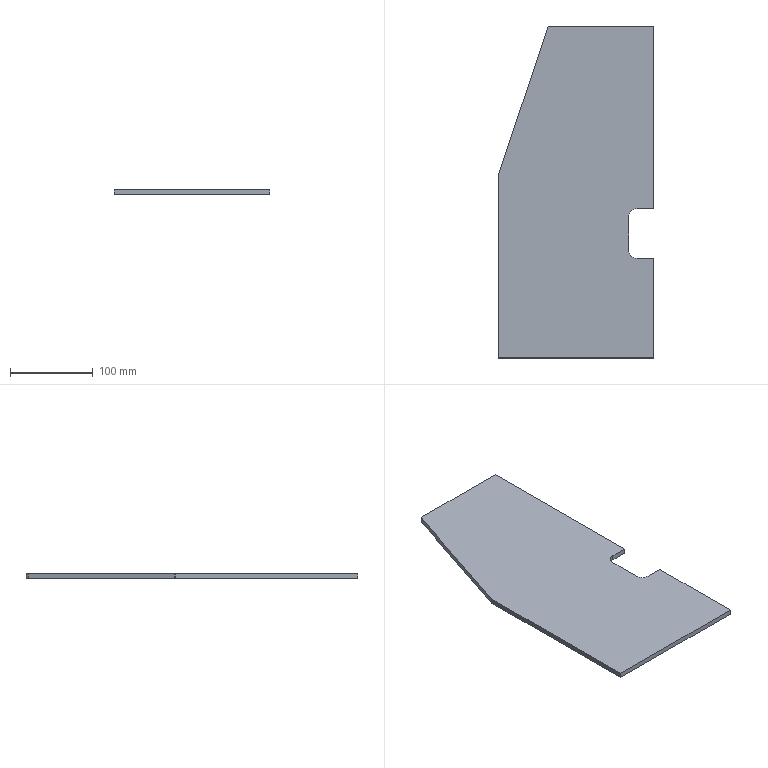Component | SolidWorks | THK-B1003LeftRearBaffle-1 | 1 solid | 15 faces | box 187 x 400 x 6 mm | volume 405848 mm3 | plane 11 | cylinder 4 | commonest cylinder face diameters 20 x2 8 x2 | material Q235A
build123d program:
from build123d import *

# Parameters (mm, degrees)
BOSS_EXTRUDE1_DEPTH = 3
CUT_EXTRUDE1_DEPTH  = 221.858
FILLET1_R           = 4


with BuildPart() as part:
    # Sketch1 → Boss-Extrude1 (new, symmetric)
    with BuildSketch(Plane(origin=(0, 0, 0), x_dir=(-1, 0, 0), z_dir=(0, 0, -1))):
        Polygon((-93.5, 200), (33.5, 200), (93.5, 20), (93.5, -200), (-93.5, -200), align=None)
    extrude(amount=BOSS_EXTRUDE1_DEPTH, both=True)

    # Sketch4 → Cut-Extrude1 (cut, through all)
    with BuildSketch(Plane.XY.offset(3)):
        with BuildLine():
            Line((73.5, -20), (93.5, -20))
            Line((93.5, -20), (93.5, -80))
            Line((93.5, -80), (73.5, -80))
            ThreePointArc((73.5, -80), (66.429, -77.071), (63.5, -70))
            Line((63.5, -70), (63.5, -30))
            ThreePointArc((63.5, -30), (66.429, -22.929), (73.5, -20))
        make_face()
    extrude(amount=-CUT_EXTRUDE1_DEPTH, mode=Mode.SUBTRACT)

    # Fillet1
    fillet1_edges = [part.edges().sort_by_distance(p)[0] for p in [
        (-33.5, 200, 0),
        (-93.5, 20, 0),
    ]]
    fillet(fillet1_edges, radius=FILLET1_R)


solid = part.part

# Placed as in the assembly
solid = solid.moved(Location((-226.5, 0, -142), (0, 0, 0)))
STEP:
#1=COLOUR_RGB('',0.7922,0.8196,0.9333);
#2=FILL_AREA_STYLE_COLOUR('',#1);
#3=FILL_AREA_STYLE('',(#2));
#4=SURFACE_STYLE_FILL_AREA(#3);
#5=SURFACE_SIDE_STYLE('',(#4));
#6=SURFACE_STYLE_USAGE(.BOTH.,#5);
#7=PRESENTATION_STYLE_ASSIGNMENT((#6));
#8=CARTESIAN_POINT('',(-5.236,-3.15,-5.709));
#9=VERTEX_POINT('',#8);
#10=CARTESIAN_POINT('',(-5.236,-7.874,-5.709));
#11=VERTEX_POINT('',#10);
#12=CARTESIAN_POINT('',(-5.236,-7.874,-5.709));
#13=DIRECTION('',(0.,-1.,0.));
#14=VECTOR('',#13,39.37);
#15=LINE('',#12,#14);
#16=EDGE_CURVE('',#9,#11,#15,.T.);
#17=ORIENTED_EDGE('',*,*,#16,.F.);
#18=CARTESIAN_POINT('',(-5.236,-3.15,-5.472));
#19=VERTEX_POINT('',#18);
#20=CARTESIAN_POINT('',(-5.236,-3.15,-5.709));
#21=DIRECTION('',(0.,0.,1.));
#22=VECTOR('',#21,39.37);
#23=LINE('',#20,#22);
#24=EDGE_CURVE('',#9,#19,#23,.T.);
#25=ORIENTED_EDGE('',*,*,#24,.T.);
#26=CARTESIAN_POINT('',(-5.236,-7.874,-5.472));
#27=VERTEX_POINT('',#26);
#28=CARTESIAN_POINT('',(-5.236,-7.874,-5.472));
#29=DIRECTION('',(0.,-1.,0.));
#30=VECTOR('',#29,39.37);
#31=LINE('',#28,#30);
#32=EDGE_CURVE('',#19,#27,#31,.T.);
#33=ORIENTED_EDGE('',*,*,#32,.T.);
#34=CARTESIAN_POINT('',(-5.236,-7.874,-5.709));
#35=DIRECTION('',(0.,0.,1.));
#36=VECTOR('',#35,39.37);
#37=LINE('',#34,#36);
#38=EDGE_CURVE('',#11,#27,#37,.T.);
#39=ORIENTED_EDGE('',*,*,#38,.F.);
#40=EDGE_LOOP('',(#17,#25,#33,#39));
#41=FACE_OUTER_BOUND('',#40,.T.);
#42=CARTESIAN_POINT('',(-5.236,-7.874,-5.709));
#43=DIRECTION('',(-1.,0.,0.));
#44=DIRECTION('',(0.,0.,1.));
#45=AXIS2_PLACEMENT_3D('',#42,#43,#44);
#46=PLANE('',#45);
#47=ADVANCED_FACE('',(#41),#46,.F.);
#48=CARTESIAN_POINT('',(-5.236,7.874,-5.472));
#49=VERTEX_POINT('',#48);
#50=CARTESIAN_POINT('',(-5.236,-0.7874,-5.472));
#51=VERTEX_POINT('',#50);
#52=CARTESIAN_POINT('',(-5.236,-7.874,-5.472));
#53=DIRECTION('',(0.,-1.,0.));
#54=VECTOR('',#53,39.37);
#55=LINE('',#52,#54);
#56=EDGE_CURVE('',#49,#51,#55,.T.);
#57=ORIENTED_EDGE('',*,*,#56,.T.);
#58=CARTESIAN_POINT('',(-5.236,-0.7874,-5.709));
#59=VERTEX_POINT('',#58);
#60=CARTESIAN_POINT('',(-5.236,-0.7874,-5.709));
#61=DIRECTION('',(0.,0.,1.));
#62=VECTOR('',#61,39.37);
#63=LINE('',#60,#62);
#64=EDGE_CURVE('',#59,#51,#63,.T.);
#65=ORIENTED_EDGE('',*,*,#64,.F.);
#66=CARTESIAN_POINT('',(-5.236,7.874,-5.709));
#67=VERTEX_POINT('',#66);
#68=CARTESIAN_POINT('',(-5.236,-7.874,-5.709));
#69=DIRECTION('',(0.,-1.,0.));
#70=VECTOR('',#69,39.37);
#71=LINE('',#68,#70);
#72=EDGE_CURVE('',#67,#59,#71,.T.);
#73=ORIENTED_EDGE('',*,*,#72,.F.);
#74=CARTESIAN_POINT('',(-5.236,7.874,-5.709));
#75=DIRECTION('',(0.,0.,1.));
#76=VECTOR('',#75,39.37);
#77=LINE('',#74,#76);
#78=EDGE_CURVE('',#67,#49,#77,.T.);
#79=ORIENTED_EDGE('',*,*,#78,.T.);
#80=EDGE_LOOP('',(#57,#65,#73,#79));
#81=FACE_OUTER_BOUND('',#80,.T.);
#82=CARTESIAN_POINT('',(-5.236,-7.874,-5.709));
#83=DIRECTION('',(-1.,0.,0.));
#84=DIRECTION('',(0.,0.,1.));
#85=AXIS2_PLACEMENT_3D('',#82,#83,#84);
#86=PLANE('',#85);
#87=ADVANCED_FACE('',(#81),#86,.F.);
#88=CARTESIAN_POINT('',(-12.598,-7.874,-5.472));
#89=VERTEX_POINT('',#88);
#90=CARTESIAN_POINT('',(-12.598,-7.874,-5.472));
#91=DIRECTION('',(-1.,0.,0.));
#92=VECTOR('',#91,39.37);
#93=LINE('',#90,#92);
#94=EDGE_CURVE('',#27,#89,#93,.T.);
#95=ORIENTED_EDGE('',*,*,#94,.T.);
#96=CARTESIAN_POINT('',(-12.598,-7.874,-5.709));
#97=VERTEX_POINT('',#96);
#98=CARTESIAN_POINT('',(-12.598,-7.874,-5.709));
#99=DIRECTION('',(0.,0.,1.));
#100=VECTOR('',#99,39.37);
#101=LINE('',#98,#100);
#102=EDGE_CURVE('',#97,#89,#101,.T.);
#103=ORIENTED_EDGE('',*,*,#102,.F.);
#104=CARTESIAN_POINT('',(-12.598,-7.874,-5.709));
#105=DIRECTION('',(-1.,0.,0.));
#106=VECTOR('',#105,39.37);
#107=LINE('',#104,#106);
#108=EDGE_CURVE('',#11,#97,#107,.T.);
#109=ORIENTED_EDGE('',*,*,#108,.F.);
#110=ORIENTED_EDGE('',*,*,#38,.T.);
#111=EDGE_LOOP('',(#95,#103,#109,#110));
#112=FACE_OUTER_BOUND('',#111,.T.);
#113=CARTESIAN_POINT('',(-12.598,-7.874,-5.709));
#114=DIRECTION('',(0.,1.,0.));
#115=DIRECTION('',(-1.,0.,0.));
#116=AXIS2_PLACEMENT_3D('',#113,#114,#115);
#117=PLANE('',#116);
#118=ADVANCED_FACE('',(#112),#117,.F.);
#119=CARTESIAN_POINT('',(-12.598,0.7618,-5.472));
#120=VERTEX_POINT('',#119);
#121=CARTESIAN_POINT('',(-12.598,0.7874,-5.472));
#122=DIRECTION('',(0.,1.,0.));
#123=VECTOR('',#122,39.37);
#124=LINE('',#121,#123);
#125=EDGE_CURVE('',#89,#120,#124,.T.);
#126=ORIENTED_EDGE('',*,*,#125,.T.);
#127=CARTESIAN_POINT('',(-12.598,0.7618,-5.709));
#128=VERTEX_POINT('',#127);
#129=CARTESIAN_POINT('',(-12.598,0.7618,-5.709));
#130=DIRECTION('',(0.,0.,-1.));
#131=VECTOR('',#130,39.37);
#132=LINE('',#129,#131);
#133=EDGE_CURVE('',#120,#128,#132,.T.);
#134=ORIENTED_EDGE('',*,*,#133,.T.);
#135=CARTESIAN_POINT('',(-12.598,0.7874,-5.709));
#136=DIRECTION('',(0.,1.,0.));
#137=VECTOR('',#136,39.37);
#138=LINE('',#135,#137);
#139=EDGE_CURVE('',#97,#128,#138,.T.);
#140=ORIENTED_EDGE('',*,*,#139,.F.);
#141=ORIENTED_EDGE('',*,*,#102,.T.);
#142=EDGE_LOOP('',(#126,#134,#140,#141));
#143=FACE_OUTER_BOUND('',#142,.T.);
#144=CARTESIAN_POINT('',(-12.598,0.7874,-5.709));
#145=DIRECTION('',(1.,-0.,0.));
#146=DIRECTION('',(0.,1.,0.));
#147=AXIS2_PLACEMENT_3D('',#144,#145,#146);
#148=PLANE('',#147);
#149=ADVANCED_FACE('',(#143),#148,.F.);
#150=CARTESIAN_POINT('',(-12.59,0.8116,-5.709));
#151=VERTEX_POINT('',#150);
#152=CARTESIAN_POINT('',(-10.272,7.766,-5.709));
#153=VERTEX_POINT('',#152);
#154=CARTESIAN_POINT('',(-10.236,7.874,-5.709));
#155=DIRECTION('',(0.3162,0.9487,0.));
#156=VECTOR('',#155,39.37);
#157=LINE('',#154,#156);
#158=EDGE_CURVE('',#151,#153,#157,.T.);
#159=ORIENTED_EDGE('',*,*,#158,.F.);
#160=CARTESIAN_POINT('',(-12.59,0.8116,-5.472));
#161=VERTEX_POINT('',#160);
#162=CARTESIAN_POINT('',(-12.59,0.8116,-5.709));
#163=DIRECTION('',(0.,0.,1.));
#164=VECTOR('',#163,39.37);
#165=LINE('',#162,#164);
#166=EDGE_CURVE('',#151,#161,#165,.T.);
#167=ORIENTED_EDGE('',*,*,#166,.T.);
#168=CARTESIAN_POINT('',(-10.272,7.766,-5.472));
#169=VERTEX_POINT('',#168);
#170=CARTESIAN_POINT('',(-10.236,7.874,-5.472));
#171=DIRECTION('',(0.3162,0.9487,0.));
#172=VECTOR('',#171,39.37);
#173=LINE('',#170,#172);
#174=EDGE_CURVE('',#161,#169,#173,.T.);
#175=ORIENTED_EDGE('',*,*,#174,.T.);
#176=CARTESIAN_POINT('',(-10.272,7.766,-5.709));
#177=DIRECTION('',(0.,0.,-1.));
#178=VECTOR('',#177,39.37);
#179=LINE('',#176,#178);
#180=EDGE_CURVE('',#169,#153,#179,.T.);
#181=ORIENTED_EDGE('',*,*,#180,.T.);
#182=EDGE_LOOP('',(#159,#167,#175,#181));
#183=FACE_OUTER_BOUND('',#182,.T.);
#184=CARTESIAN_POINT('',(-10.236,7.874,-5.709));
#185=DIRECTION('',(0.9487,-0.3162,0.));
#186=DIRECTION('',(0.3162,0.9487,0.));
#187=AXIS2_PLACEMENT_3D('',#184,#185,#186);
#188=PLANE('',#187);
#189=ADVANCED_FACE('',(#183),#188,.F.);
#190=CARTESIAN_POINT('',(-10.123,7.874,-5.709));
#191=VERTEX_POINT('',#190);
#192=CARTESIAN_POINT('',(-5.236,7.874,-5.709));
#193=DIRECTION('',(1.,0.,0.));
#194=VECTOR('',#193,39.37);
#195=LINE('',#192,#194);
#196=EDGE_CURVE('',#191,#67,#195,.T.);
#197=ORIENTED_EDGE('',*,*,#196,.F.);
#198=CARTESIAN_POINT('',(-10.123,7.874,-5.472));
#199=VERTEX_POINT('',#198);
#200=CARTESIAN_POINT('',(-10.123,7.874,-5.709));
#201=DIRECTION('',(0.,0.,1.));
#202=VECTOR('',#201,39.37);
#203=LINE('',#200,#202);
#204=EDGE_CURVE('',#191,#199,#203,.T.);
#205=ORIENTED_EDGE('',*,*,#204,.T.);
#206=CARTESIAN_POINT('',(-5.236,7.874,-5.472));
#207=DIRECTION('',(1.,0.,0.));
#208=VECTOR('',#207,39.37);
#209=LINE('',#206,#208);
#210=EDGE_CURVE('',#199,#49,#209,.T.);
#211=ORIENTED_EDGE('',*,*,#210,.T.);
#212=ORIENTED_EDGE('',*,*,#78,.F.);
#213=EDGE_LOOP('',(#197,#205,#211,#212));
#214=FACE_OUTER_BOUND('',#213,.T.);
#215=CARTESIAN_POINT('',(-5.236,7.874,-5.709));
#216=DIRECTION('',(0.,-1.,0.));
#217=DIRECTION('',(0.,0.,-1.));
#218=AXIS2_PLACEMENT_3D('',#215,#216,#217);
#219=PLANE('',#218);
#220=ADVANCED_FACE('',(#214),#219,.F.);
#221=ORIENTED_EDGE('',*,*,#139,.T.);
#222=CARTESIAN_POINT('',(-12.441,0.7618,-5.709));
#223=DIRECTION('',(0.,0.,-1.));
#224=DIRECTION('',(1.,0.,0.));
#225=AXIS2_PLACEMENT_3D('',#222,#223,#224);
#226=CIRCLE('',#225,0.1575);
#227=EDGE_CURVE('',#128,#151,#226,.T.);
#228=ORIENTED_EDGE('',*,*,#227,.T.);
#229=ORIENTED_EDGE('',*,*,#158,.T.);
#230=CARTESIAN_POINT('',(-10.123,7.717,-5.709));
#231=DIRECTION('',(0.,0.,-1.));
#232=DIRECTION('',(1.,0.,0.));
#233=AXIS2_PLACEMENT_3D('',#230,#231,#232);
#234=CIRCLE('',#233,0.1575);
#235=EDGE_CURVE('',#153,#191,#234,.T.);
#236=ORIENTED_EDGE('',*,*,#235,.T.);
#237=ORIENTED_EDGE('',*,*,#196,.T.);
#238=ORIENTED_EDGE('',*,*,#72,.T.);
#239=CARTESIAN_POINT('',(-6.024,-0.7874,-5.709));
#240=VERTEX_POINT('',#239);
#241=CARTESIAN_POINT('',(-6.024,-0.7874,-5.709));
#242=DIRECTION('',(-1.,0.,0.));
#243=VECTOR('',#242,39.37);
#244=LINE('',#241,#243);
#245=EDGE_CURVE('',#59,#240,#244,.T.);
#246=ORIENTED_EDGE('',*,*,#245,.T.);
#247=CARTESIAN_POINT('',(-6.417,-1.181,-5.709));
#248=VERTEX_POINT('',#247);
#249=CARTESIAN_POINT('',(-6.024,-1.181,-5.709));
#250=DIRECTION('',(0.,0.,1.));
#251=DIRECTION('',(-1.,0.,0.));
#252=AXIS2_PLACEMENT_3D('',#249,#250,#251);
#253=CIRCLE('',#252,0.3937);
#254=EDGE_CURVE('',#240,#248,#253,.T.);
#255=ORIENTED_EDGE('',*,*,#254,.T.);
#256=CARTESIAN_POINT('',(-6.417,-2.756,-5.709));
#257=VERTEX_POINT('',#256);
#258=CARTESIAN_POINT('',(-6.417,-1.181,-5.709));
#259=DIRECTION('',(0.,-1.,0.));
#260=VECTOR('',#259,39.37);
#261=LINE('',#258,#260);
#262=EDGE_CURVE('',#248,#257,#261,.T.);
#263=ORIENTED_EDGE('',*,*,#262,.T.);
#264=CARTESIAN_POINT('',(-6.024,-3.15,-5.709));
#265=VERTEX_POINT('',#264);
#266=CARTESIAN_POINT('',(-6.024,-2.756,-5.709));
#267=DIRECTION('',(0.,0.,1.));
#268=DIRECTION('',(1.,0.,0.));
#269=AXIS2_PLACEMENT_3D('',#266,#267,#268);
#270=CIRCLE('',#269,0.3937);
#271=EDGE_CURVE('',#257,#265,#270,.T.);
#272=ORIENTED_EDGE('',*,*,#271,.T.);
#273=CARTESIAN_POINT('',(-6.024,-3.15,-5.709));
#274=DIRECTION('',(1.,0.,0.));
#275=VECTOR('',#274,39.37);
#276=LINE('',#273,#275);
#277=EDGE_CURVE('',#265,#9,#276,.T.);
#278=ORIENTED_EDGE('',*,*,#277,.T.);
#279=ORIENTED_EDGE('',*,*,#16,.T.);
#280=ORIENTED_EDGE('',*,*,#108,.T.);
#281=EDGE_LOOP('',(#221,#228,#229,#236,#237,#238,#246,#255,#263,#272,#278,#279,#280));
#282=FACE_OUTER_BOUND('',#281,.T.);
#283=CARTESIAN_POINT('',(-8.917,0.,-5.709));
#284=DIRECTION('',(0.,0.,1.));
#285=DIRECTION('',(1.,0.,0.));
#286=AXIS2_PLACEMENT_3D('',#283,#284,#285);
#287=PLANE('',#286);
#288=ADVANCED_FACE('',(#282),#287,.F.);
#289=ORIENTED_EDGE('',*,*,#174,.F.);
#290=CARTESIAN_POINT('',(-12.441,0.7618,-5.472));
#291=DIRECTION('',(0.,0.,1.));
#292=DIRECTION('',(1.,0.,0.));
#293=AXIS2_PLACEMENT_3D('',#290,#291,#292);
#294=CIRCLE('',#293,0.1575);
#295=EDGE_CURVE('',#161,#120,#294,.T.);
#296=ORIENTED_EDGE('',*,*,#295,.T.);
#297=ORIENTED_EDGE('',*,*,#125,.F.);
#298=ORIENTED_EDGE('',*,*,#94,.F.);
#299=ORIENTED_EDGE('',*,*,#32,.F.);
#300=CARTESIAN_POINT('',(-6.024,-3.15,-5.472));
#301=VERTEX_POINT('',#300);
#302=CARTESIAN_POINT('',(-6.024,-3.15,-5.472));
#303=DIRECTION('',(1.,0.,0.));
#304=VECTOR('',#303,39.37);
#305=LINE('',#302,#304);
#306=EDGE_CURVE('',#301,#19,#305,.T.);
#307=ORIENTED_EDGE('',*,*,#306,.F.);
#308=CARTESIAN_POINT('',(-6.417,-2.756,-5.472));
#309=VERTEX_POINT('',#308);
#310=CARTESIAN_POINT('',(-6.024,-2.756,-5.472));
#311=DIRECTION('',(0.,0.,1.));
#312=DIRECTION('',(1.,0.,0.));
#313=AXIS2_PLACEMENT_3D('',#310,#311,#312);
#314=CIRCLE('',#313,0.3937);
#315=EDGE_CURVE('',#309,#301,#314,.T.);
#316=ORIENTED_EDGE('',*,*,#315,.F.);
#317=CARTESIAN_POINT('',(-6.417,-1.181,-5.472));
#318=VERTEX_POINT('',#317);
#319=CARTESIAN_POINT('',(-6.417,-1.181,-5.472));
#320=DIRECTION('',(0.,-1.,0.));
#321=VECTOR('',#320,39.37);
#322=LINE('',#319,#321);
#323=EDGE_CURVE('',#318,#309,#322,.T.);
#324=ORIENTED_EDGE('',*,*,#323,.F.);
#325=CARTESIAN_POINT('',(-6.024,-0.7874,-5.472));
#326=VERTEX_POINT('',#325);
#327=CARTESIAN_POINT('',(-6.024,-1.181,-5.472));
#328=DIRECTION('',(0.,0.,1.));
#329=DIRECTION('',(-1.,0.,0.));
#330=AXIS2_PLACEMENT_3D('',#327,#328,#329);
#331=CIRCLE('',#330,0.3937);
#332=EDGE_CURVE('',#326,#318,#331,.T.);
#333=ORIENTED_EDGE('',*,*,#332,.F.);
#334=CARTESIAN_POINT('',(-6.024,-0.7874,-5.472));
#335=DIRECTION('',(-1.,0.,0.));
#336=VECTOR('',#335,39.37);
#337=LINE('',#334,#336);
#338=EDGE_CURVE('',#51,#326,#337,.T.);
#339=ORIENTED_EDGE('',*,*,#338,.F.);
#340=ORIENTED_EDGE('',*,*,#56,.F.);
#341=ORIENTED_EDGE('',*,*,#210,.F.);
#342=CARTESIAN_POINT('',(-10.123,7.717,-5.472));
#343=DIRECTION('',(0.,0.,1.));
#344=DIRECTION('',(1.,0.,0.));
#345=AXIS2_PLACEMENT_3D('',#342,#343,#344);
#346=CIRCLE('',#345,0.1575);
#347=EDGE_CURVE('',#199,#169,#346,.T.);
#348=ORIENTED_EDGE('',*,*,#347,.T.);
#349=EDGE_LOOP('',(#289,#296,#297,#298,#299,#307,#316,#324,#333,#339,#340,#341,#348));
#350=FACE_OUTER_BOUND('',#349,.T.);
#351=CARTESIAN_POINT('',(-8.917,0.,-5.472));
#352=DIRECTION('',(0.,0.,1.));
#353=DIRECTION('',(1.,0.,0.));
#354=AXIS2_PLACEMENT_3D('',#351,#352,#353);
#355=PLANE('',#354);
#356=ADVANCED_FACE('',(#350),#355,.T.);
#357=ORIENTED_EDGE('',*,*,#306,.T.);
#358=ORIENTED_EDGE('',*,*,#24,.F.);
#359=ORIENTED_EDGE('',*,*,#277,.F.);
#360=CARTESIAN_POINT('',(-6.024,-3.15,-5.709));
#361=DIRECTION('',(0.,0.,1.));
#362=VECTOR('',#361,39.37);
#363=LINE('',#360,#362);
#364=EDGE_CURVE('',#265,#301,#363,.T.);
#365=ORIENTED_EDGE('',*,*,#364,.T.);
#366=EDGE_LOOP('',(#357,#358,#359,#365));
#367=FACE_OUTER_BOUND('',#366,.T.);
#368=CARTESIAN_POINT('',(-6.024,-3.15,-5.709));
#369=DIRECTION('',(0.,-1.,0.));
#370=DIRECTION('',(0.,0.,-1.));
#371=AXIS2_PLACEMENT_3D('',#368,#369,#370);
#372=PLANE('',#371);
#373=ADVANCED_FACE('',(#367),#372,.F.);
#374=ORIENTED_EDGE('',*,*,#315,.T.);
#375=ORIENTED_EDGE('',*,*,#364,.F.);
#376=ORIENTED_EDGE('',*,*,#271,.F.);
#377=CARTESIAN_POINT('',(-6.417,-2.756,-5.709));
#378=DIRECTION('',(0.,0.,1.));
#379=VECTOR('',#378,39.37);
#380=LINE('',#377,#379);
#381=EDGE_CURVE('',#257,#309,#380,.T.);
#382=ORIENTED_EDGE('',*,*,#381,.T.);
#383=EDGE_LOOP('',(#374,#375,#376,#382));
#384=FACE_OUTER_BOUND('',#383,.T.);
#385=CARTESIAN_POINT('',(-6.024,-2.756,-5.709));
#386=DIRECTION('',(0.,0.,1.));
#387=DIRECTION('',(1.,0.,0.));
#388=AXIS2_PLACEMENT_3D('',#385,#386,#387);
#389=CYLINDRICAL_SURFACE('',#388,0.3937);
#390=ADVANCED_FACE('',(#384),#389,.F.);
#391=ORIENTED_EDGE('',*,*,#323,.T.);
#392=ORIENTED_EDGE('',*,*,#381,.F.);
#393=ORIENTED_EDGE('',*,*,#262,.F.);
#394=CARTESIAN_POINT('',(-6.417,-1.181,-5.709));
#395=DIRECTION('',(0.,0.,1.));
#396=VECTOR('',#395,39.37);
#397=LINE('',#394,#396);
#398=EDGE_CURVE('',#248,#318,#397,.T.);
#399=ORIENTED_EDGE('',*,*,#398,.T.);
#400=EDGE_LOOP('',(#391,#392,#393,#399));
#401=FACE_OUTER_BOUND('',#400,.T.);
#402=CARTESIAN_POINT('',(-6.417,-1.181,-5.709));
#403=DIRECTION('',(-1.,0.,0.));
#404=DIRECTION('',(0.,0.,1.));
#405=AXIS2_PLACEMENT_3D('',#402,#403,#404);
#406=PLANE('',#405);
#407=ADVANCED_FACE('',(#401),#406,.F.);
#408=ORIENTED_EDGE('',*,*,#332,.T.);
#409=ORIENTED_EDGE('',*,*,#398,.F.);
#410=ORIENTED_EDGE('',*,*,#254,.F.);
#411=CARTESIAN_POINT('',(-6.024,-0.7874,-5.709));
#412=DIRECTION('',(0.,0.,1.));
#413=VECTOR('',#412,39.37);
#414=LINE('',#411,#413);
#415=EDGE_CURVE('',#240,#326,#414,.T.);
#416=ORIENTED_EDGE('',*,*,#415,.T.);
#417=EDGE_LOOP('',(#408,#409,#410,#416));
#418=FACE_OUTER_BOUND('',#417,.T.);
#419=CARTESIAN_POINT('',(-6.024,-1.181,-5.709));
#420=DIRECTION('',(0.,0.,1.));
#421=DIRECTION('',(1.,0.,0.));
#422=AXIS2_PLACEMENT_3D('',#419,#420,#421);
#423=CYLINDRICAL_SURFACE('',#422,0.3937);
#424=ADVANCED_FACE('',(#418),#423,.F.);
#425=ORIENTED_EDGE('',*,*,#338,.T.);
#426=ORIENTED_EDGE('',*,*,#415,.F.);
#427=ORIENTED_EDGE('',*,*,#245,.F.);
#428=ORIENTED_EDGE('',*,*,#64,.T.);
#429=EDGE_LOOP('',(#425,#426,#427,#428));
#430=FACE_OUTER_BOUND('',#429,.T.);
#431=CARTESIAN_POINT('',(-6.024,-0.7874,-5.709));
#432=DIRECTION('',(0.,1.,0.));
#433=DIRECTION('',(-1.,0.,0.));
#434=AXIS2_PLACEMENT_3D('',#431,#432,#433);
#435=PLANE('',#434);
#436=ADVANCED_FACE('',(#430),#435,.F.);
#437=ORIENTED_EDGE('',*,*,#227,.F.);
#438=ORIENTED_EDGE('',*,*,#133,.F.);
#439=ORIENTED_EDGE('',*,*,#295,.F.);
#440=ORIENTED_EDGE('',*,*,#166,.F.);
#441=EDGE_LOOP('',(#437,#438,#439,#440));
#442=FACE_OUTER_BOUND('',#441,.T.);
#443=CARTESIAN_POINT('',(-12.441,0.7618,-5.709));
#444=DIRECTION('',(0.,0.,1.));
#445=DIRECTION('',(1.,0.,0.));
#446=AXIS2_PLACEMENT_3D('',#443,#444,#445);
#447=CYLINDRICAL_SURFACE('',#446,0.1575);
#448=ADVANCED_FACE('',(#442),#447,.T.);
#449=ORIENTED_EDGE('',*,*,#235,.F.);
#450=ORIENTED_EDGE('',*,*,#180,.F.);
#451=ORIENTED_EDGE('',*,*,#347,.F.);
#452=ORIENTED_EDGE('',*,*,#204,.F.);
#453=EDGE_LOOP('',(#449,#450,#451,#452));
#454=FACE_OUTER_BOUND('',#453,.T.);
#455=CARTESIAN_POINT('',(-10.123,7.717,-5.709));
#456=DIRECTION('',(0.,0.,1.));
#457=DIRECTION('',(1.,0.,0.));
#458=AXIS2_PLACEMENT_3D('',#455,#456,#457);
#459=CYLINDRICAL_SURFACE('',#458,0.1575);
#460=ADVANCED_FACE('',(#454),#459,.T.);
#461=CLOSED_SHELL('',(#47,#87,#118,#149,#189,#220,#288,#356,#373,#390,#407,#424,#436,#448,#460));
#462=MANIFOLD_SOLID_BREP('',#461);
#463=STYLED_ITEM('',(#7),#462);
#464=PRESENTATION_LAYER_ASSIGNMENT('','',(#463));
#465=(LENGTH_UNIT()NAMED_UNIT(*)SI_UNIT($,.METRE.));
#466=LENGTH_MEASURE_WITH_UNIT(LENGTH_MEASURE(0.0254),#465);
#467=DIMENSIONAL_EXPONENTS(1.,0.,0.,0.,0.,0.,0.);
#468=(CONVERSION_BASED_UNIT('',#466)LENGTH_UNIT()NAMED_UNIT(#467));
#469=UNCERTAINTY_MEASURE_WITH_UNIT(LENGTH_MEASURE(0.00001),#468,'','');
#470=(NAMED_UNIT(*)PLANE_ANGLE_UNIT()SI_UNIT($,.RADIAN.));
#471=(NAMED_UNIT(*)SI_UNIT($,.STERADIAN.)SOLID_ANGLE_UNIT());
#472=(GEOMETRIC_REPRESENTATION_CONTEXT(3)GLOBAL_UNCERTAINTY_ASSIGNED_CONTEXT((#469))GLOBAL_UNIT_ASSIGNED_CONTEXT((#468,#470,#471))REPRESENTATION_CONTEXT('',''));
#473=MECHANICAL_DESIGN_GEOMETRIC_PRESENTATION_REPRESENTATION('',(#463),#472);
#474=CARTESIAN_POINT('',(0.,0.,0.));
#475=DIRECTION('',(0.,0.,1.));
#476=DIRECTION('',(1.,0.,0.));
#477=AXIS2_PLACEMENT_3D('',#474,#475,#476);
#478=(LENGTH_UNIT()NAMED_UNIT(*)SI_UNIT($,.METRE.));
#479=LENGTH_MEASURE_WITH_UNIT(LENGTH_MEASURE(0.0254),#478);
#480=DIMENSIONAL_EXPONENTS(1.,0.,0.,0.,0.,0.,0.);
#481=(CONVERSION_BASED_UNIT('',#479)LENGTH_UNIT()NAMED_UNIT(#480));
#482=UNCERTAINTY_MEASURE_WITH_UNIT(LENGTH_MEASURE(0.00001),#481,'','');
#483=(NAMED_UNIT(*)PLANE_ANGLE_UNIT()SI_UNIT($,.RADIAN.));
#484=(NAMED_UNIT(*)SI_UNIT($,.STERADIAN.)SOLID_ANGLE_UNIT());
#485=(GEOMETRIC_REPRESENTATION_CONTEXT(3)GLOBAL_UNCERTAINTY_ASSIGNED_CONTEXT((#482))GLOBAL_UNIT_ASSIGNED_CONTEXT((#481,#483,#484))REPRESENTATION_CONTEXT('',''));
#486=ADVANCED_BREP_SHAPE_REPRESENTATION('',(#462,#477),#485);